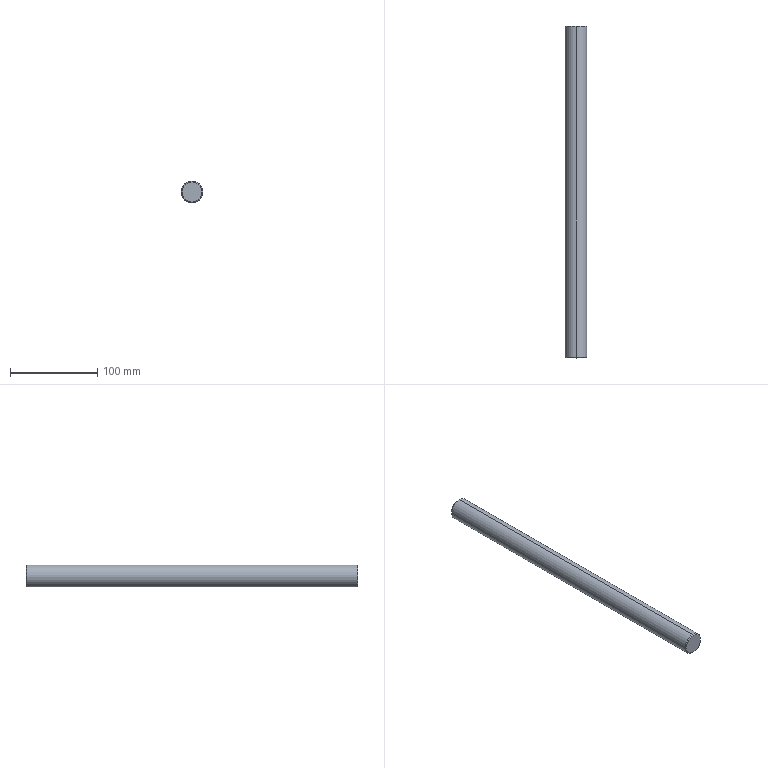Component | SolidWorks | 8TC-A15004-90-02A-1 | 1 solid | 8 faces | box 25 x 380 x 25 mm | volume 186456 mm3 | cone 4 | cylinder 2 | plane 2 | commonest cylinder face diameters 25 x2 | material Chrome Plated Rod
build123d program:
from build123d import *

# Parameters (mm, degrees)
SKETCH1_R           = 12.5
BOSS_EXTRUDE1_DEPTH = 190
CHAMFER1_SIZE       = 1


with BuildPart() as part:
    # Sketch1 → Boss-Extrude1 (new, symmetric)
    with BuildSketch(Plane(origin=(0, 0, 0), x_dir=(0, 0, -1), z_dir=(1, 0, 0))):
        Circle(SKETCH1_R)
    extrude(amount=BOSS_EXTRUDE1_DEPTH, both=True)

    # Chamfer1
    chamfer1_edges = [part.edges().sort_by_distance(p)[0] for p in [
        (-190, 0, 12.5),
        (190, 0, 12.5),
    ]]
    chamfer(chamfer1_edges, length=CHAMFER1_SIZE)


solid = part.part

# Placed as in the assembly
solid = solid.moved(Location((-15, 180, 0), (0, 0, 90)))
STEP:
#1=COLOUR_RGB('',0.7922,0.8196,0.9333);
#2=FILL_AREA_STYLE_COLOUR('',#1);
#3=FILL_AREA_STYLE('',(#2));
#4=SURFACE_STYLE_FILL_AREA(#3);
#5=SURFACE_SIDE_STYLE('',(#4));
#6=SURFACE_STYLE_USAGE(.BOTH.,#5);
#7=PRESENTATION_STYLE_ASSIGNMENT((#6));
#8=CARTESIAN_POINT('',(-0.5906,-0.3937,-0.4528));
#9=VERTEX_POINT('',#8);
#10=CARTESIAN_POINT('',(-0.5906,-0.3937,0.4528));
#11=VERTEX_POINT('',#10);
#12=CARTESIAN_POINT('',(-0.5906,-0.3937,0.));
#13=DIRECTION('',(0.,-1.,0.));
#14=DIRECTION('',(0.,0.,-1.));
#15=AXIS2_PLACEMENT_3D('',#12,#13,#14);
#16=CIRCLE('',#15,0.4528);
#17=EDGE_CURVE('',#9,#11,#16,.T.);
#18=ORIENTED_EDGE('',*,*,#17,.F.);
#19=CARTESIAN_POINT('',(-0.5906,-0.3543,-0.4921));
#20=VERTEX_POINT('',#19);
#21=CARTESIAN_POINT('',(-0.5906,-0.3937,-0.4528));
#22=DIRECTION('',(0.,0.7071,-0.7071));
#23=VECTOR('',#22,39.37);
#24=LINE('',#21,#23);
#25=EDGE_CURVE('',#9,#20,#24,.T.);
#26=ORIENTED_EDGE('',*,*,#25,.T.);
#27=CARTESIAN_POINT('',(-0.5906,-0.3543,0.4921));
#28=VERTEX_POINT('',#27);
#29=CARTESIAN_POINT('',(-0.5906,-0.3543,0.));
#30=DIRECTION('',(0.,1.,0.));
#31=DIRECTION('',(0.,0.,-1.));
#32=AXIS2_PLACEMENT_3D('',#29,#30,#31);
#33=CIRCLE('',#32,0.4921);
#34=EDGE_CURVE('',#28,#20,#33,.T.);
#35=ORIENTED_EDGE('',*,*,#34,.F.);
#36=CARTESIAN_POINT('',(-0.5906,-0.3937,0.4528));
#37=DIRECTION('',(0.,0.7071,0.7071));
#38=VECTOR('',#37,39.37);
#39=LINE('',#36,#38);
#40=EDGE_CURVE('',#11,#28,#39,.T.);
#41=ORIENTED_EDGE('',*,*,#40,.F.);
#42=EDGE_LOOP('',(#18,#26,#35,#41));
#43=FACE_OUTER_BOUND('',#42,.T.);
#44=CARTESIAN_POINT('',(-0.5906,-0.3937,0.));
#45=DIRECTION('',(0.,1.,0.));
#46=DIRECTION('',(0.,0.,1.));
#47=AXIS2_PLACEMENT_3D('',#44,#45,#46);
#48=CONICAL_SURFACE('',#47,0.4528,0.7854);
#49=ADVANCED_FACE('',(#43),#48,.T.);
#50=CARTESIAN_POINT('',(-0.5906,14.567,0.4528));
#51=VERTEX_POINT('',#50);
#52=CARTESIAN_POINT('',(-0.5906,14.567,-0.4528));
#53=VERTEX_POINT('',#52);
#54=CARTESIAN_POINT('',(-0.5906,14.567,0.));
#55=DIRECTION('',(0.,1.,0.));
#56=DIRECTION('',(0.,0.,-1.));
#57=AXIS2_PLACEMENT_3D('',#54,#55,#56);
#58=CIRCLE('',#57,0.4528);
#59=EDGE_CURVE('',#51,#53,#58,.T.);
#60=ORIENTED_EDGE('',*,*,#59,.F.);
#61=CARTESIAN_POINT('',(-0.5906,14.528,0.4921));
#62=VERTEX_POINT('',#61);
#63=CARTESIAN_POINT('',(-0.5906,14.528,0.4921));
#64=DIRECTION('',(0.,-0.7071,0.7071));
#65=VECTOR('',#64,39.37);
#66=LINE('',#63,#65);
#67=EDGE_CURVE('',#51,#62,#66,.T.);
#68=ORIENTED_EDGE('',*,*,#67,.T.);
#69=CARTESIAN_POINT('',(-0.5906,14.528,-0.4921));
#70=VERTEX_POINT('',#69);
#71=CARTESIAN_POINT('',(-0.5906,14.528,0.));
#72=DIRECTION('',(0.,-1.,0.));
#73=DIRECTION('',(0.,0.,-1.));
#74=AXIS2_PLACEMENT_3D('',#71,#72,#73);
#75=CIRCLE('',#74,0.4921);
#76=EDGE_CURVE('',#70,#62,#75,.T.);
#77=ORIENTED_EDGE('',*,*,#76,.F.);
#78=CARTESIAN_POINT('',(-0.5906,14.528,-0.4921));
#79=DIRECTION('',(0.,-0.7071,-0.7071));
#80=VECTOR('',#79,39.37);
#81=LINE('',#78,#80);
#82=EDGE_CURVE('',#53,#70,#81,.T.);
#83=ORIENTED_EDGE('',*,*,#82,.F.);
#84=EDGE_LOOP('',(#60,#68,#77,#83));
#85=FACE_OUTER_BOUND('',#84,.T.);
#86=CARTESIAN_POINT('',(-0.5906,14.528,0.));
#87=DIRECTION('',(0.,-1.,0.));
#88=DIRECTION('',(0.,0.,-1.));
#89=AXIS2_PLACEMENT_3D('',#86,#87,#88);
#90=CONICAL_SURFACE('',#89,0.4921,0.7854);
#91=ADVANCED_FACE('',(#85),#90,.T.);
#92=ORIENTED_EDGE('',*,*,#34,.T.);
#93=CARTESIAN_POINT('',(-0.5906,-0.3937,-0.4921));
#94=DIRECTION('',(0.,1.,0.));
#95=VECTOR('',#94,39.37);
#96=LINE('',#93,#95);
#97=EDGE_CURVE('',#20,#70,#96,.T.);
#98=ORIENTED_EDGE('',*,*,#97,.T.);
#99=ORIENTED_EDGE('',*,*,#76,.T.);
#100=CARTESIAN_POINT('',(-0.5906,-0.3937,0.4921));
#101=DIRECTION('',(0.,1.,0.));
#102=VECTOR('',#101,39.37);
#103=LINE('',#100,#102);
#104=EDGE_CURVE('',#28,#62,#103,.T.);
#105=ORIENTED_EDGE('',*,*,#104,.F.);
#106=EDGE_LOOP('',(#92,#98,#99,#105));
#107=FACE_OUTER_BOUND('',#106,.T.);
#108=CARTESIAN_POINT('',(-0.5906,-0.3937,0.));
#109=DIRECTION('',(0.,1.,0.));
#110=DIRECTION('',(0.,0.,1.));
#111=AXIS2_PLACEMENT_3D('',#108,#109,#110);
#112=CYLINDRICAL_SURFACE('',#111,0.4921);
#113=ADVANCED_FACE('',(#107),#112,.T.);
#114=ORIENTED_EDGE('',*,*,#97,.F.);
#115=CARTESIAN_POINT('',(-0.5906,-0.3543,0.));
#116=DIRECTION('',(0.,1.,0.));
#117=DIRECTION('',(0.,0.,-1.));
#118=AXIS2_PLACEMENT_3D('',#115,#116,#117);
#119=CIRCLE('',#118,0.4921);
#120=EDGE_CURVE('',#20,#28,#119,.T.);
#121=ORIENTED_EDGE('',*,*,#120,.T.);
#122=ORIENTED_EDGE('',*,*,#104,.T.);
#123=CARTESIAN_POINT('',(-0.5906,14.528,0.));
#124=DIRECTION('',(0.,-1.,0.));
#125=DIRECTION('',(0.,0.,-1.));
#126=AXIS2_PLACEMENT_3D('',#123,#124,#125);
#127=CIRCLE('',#126,0.4921);
#128=EDGE_CURVE('',#62,#70,#127,.T.);
#129=ORIENTED_EDGE('',*,*,#128,.T.);
#130=EDGE_LOOP('',(#114,#121,#122,#129));
#131=FACE_OUTER_BOUND('',#130,.T.);
#132=CARTESIAN_POINT('',(-0.5906,-0.3937,0.));
#133=DIRECTION('',(0.,1.,0.));
#134=DIRECTION('',(0.,0.,1.));
#135=AXIS2_PLACEMENT_3D('',#132,#133,#134);
#136=CYLINDRICAL_SURFACE('',#135,0.4921);
#137=ADVANCED_FACE('',(#131),#136,.T.);
#138=CARTESIAN_POINT('',(-0.5906,-0.3937,0.));
#139=DIRECTION('',(0.,-1.,0.));
#140=DIRECTION('',(0.,0.,-1.));
#141=AXIS2_PLACEMENT_3D('',#138,#139,#140);
#142=CIRCLE('',#141,0.4528);
#143=EDGE_CURVE('',#11,#9,#142,.T.);
#144=ORIENTED_EDGE('',*,*,#143,.T.);
#145=ORIENTED_EDGE('',*,*,#17,.T.);
#146=EDGE_LOOP('',(#144,#145));
#147=FACE_OUTER_BOUND('',#146,.T.);
#148=CARTESIAN_POINT('',(-0.5906,-0.3937,0.));
#149=DIRECTION('',(0.,-1.,0.));
#150=DIRECTION('',(0.,0.,-1.));
#151=AXIS2_PLACEMENT_3D('',#148,#149,#150);
#152=PLANE('',#151);
#153=ADVANCED_FACE('',(#147),#152,.T.);
#154=CARTESIAN_POINT('',(-0.5906,14.567,0.));
#155=DIRECTION('',(0.,1.,0.));
#156=DIRECTION('',(0.,0.,-1.));
#157=AXIS2_PLACEMENT_3D('',#154,#155,#156);
#158=CIRCLE('',#157,0.4528);
#159=EDGE_CURVE('',#53,#51,#158,.T.);
#160=ORIENTED_EDGE('',*,*,#159,.T.);
#161=ORIENTED_EDGE('',*,*,#59,.T.);
#162=EDGE_LOOP('',(#160,#161));
#163=FACE_OUTER_BOUND('',#162,.T.);
#164=CARTESIAN_POINT('',(-0.5906,14.567,0.));
#165=DIRECTION('',(0.,-1.,0.));
#166=DIRECTION('',(0.,0.,-1.));
#167=AXIS2_PLACEMENT_3D('',#164,#165,#166);
#168=PLANE('',#167);
#169=ADVANCED_FACE('',(#163),#168,.F.);
#170=ORIENTED_EDGE('',*,*,#67,.F.);
#171=ORIENTED_EDGE('',*,*,#159,.F.);
#172=ORIENTED_EDGE('',*,*,#82,.T.);
#173=ORIENTED_EDGE('',*,*,#128,.F.);
#174=EDGE_LOOP('',(#170,#171,#172,#173));
#175=FACE_OUTER_BOUND('',#174,.T.);
#176=CARTESIAN_POINT('',(-0.5906,14.528,0.));
#177=DIRECTION('',(0.,-1.,0.));
#178=DIRECTION('',(0.,0.,-1.));
#179=AXIS2_PLACEMENT_3D('',#176,#177,#178);
#180=CONICAL_SURFACE('',#179,0.4921,0.7854);
#181=ADVANCED_FACE('',(#175),#180,.T.);
#182=ORIENTED_EDGE('',*,*,#25,.F.);
#183=ORIENTED_EDGE('',*,*,#143,.F.);
#184=ORIENTED_EDGE('',*,*,#40,.T.);
#185=ORIENTED_EDGE('',*,*,#120,.F.);
#186=EDGE_LOOP('',(#182,#183,#184,#185));
#187=FACE_OUTER_BOUND('',#186,.T.);
#188=CARTESIAN_POINT('',(-0.5906,-0.3937,0.));
#189=DIRECTION('',(0.,1.,0.));
#190=DIRECTION('',(0.,0.,1.));
#191=AXIS2_PLACEMENT_3D('',#188,#189,#190);
#192=CONICAL_SURFACE('',#191,0.4528,0.7854);
#193=ADVANCED_FACE('',(#187),#192,.T.);
#194=CLOSED_SHELL('',(#49,#91,#113,#137,#153,#169,#181,#193));
#195=MANIFOLD_SOLID_BREP('',#194);
#196=STYLED_ITEM('',(#7),#195);
#197=PRESENTATION_LAYER_ASSIGNMENT('','',(#196));
#198=CARTESIAN_POINT('',(0.,0.,0.));
#199=DIRECTION('',(0.,0.,1.));
#200=DIRECTION('',(1.,0.,0.));
#201=AXIS2_PLACEMENT_3D('',#198,#199,#200);
#202=(LENGTH_UNIT()NAMED_UNIT(*)SI_UNIT($,.METRE.));
#203=LENGTH_MEASURE_WITH_UNIT(LENGTH_MEASURE(0.0254),#202);
#204=DIMENSIONAL_EXPONENTS(1.,0.,0.,0.,0.,0.,0.);
#205=(CONVERSION_BASED_UNIT('',#203)LENGTH_UNIT()NAMED_UNIT(#204));
#206=UNCERTAINTY_MEASURE_WITH_UNIT(LENGTH_MEASURE(0.00001),#205,'','');
#207=(NAMED_UNIT(*)PLANE_ANGLE_UNIT()SI_UNIT($,.RADIAN.));
#208=(NAMED_UNIT(*)SI_UNIT($,.STERADIAN.)SOLID_ANGLE_UNIT());
#209=(GEOMETRIC_REPRESENTATION_CONTEXT(3)GLOBAL_UNCERTAINTY_ASSIGNED_CONTEXT((#206))GLOBAL_UNIT_ASSIGNED_CONTEXT((#205,#207,#208))REPRESENTATION_CONTEXT('',''));
#210=ADVANCED_BREP_SHAPE_REPRESENTATION('',(#195,#201),#209);
#211=(LENGTH_UNIT()NAMED_UNIT(*)SI_UNIT($,.METRE.));
#212=LENGTH_MEASURE_WITH_UNIT(LENGTH_MEASURE(0.0254),#211);
#213=DIMENSIONAL_EXPONENTS(1.,0.,0.,0.,0.,0.,0.);
#214=(CONVERSION_BASED_UNIT('',#212)LENGTH_UNIT()NAMED_UNIT(#213));
#215=UNCERTAINTY_MEASURE_WITH_UNIT(LENGTH_MEASURE(0.00001),#214,'','');
#216=(NAMED_UNIT(*)PLANE_ANGLE_UNIT()SI_UNIT($,.RADIAN.));
#217=(NAMED_UNIT(*)SI_UNIT($,.STERADIAN.)SOLID_ANGLE_UNIT());
#218=(GEOMETRIC_REPRESENTATION_CONTEXT(3)GLOBAL_UNCERTAINTY_ASSIGNED_CONTEXT((#215))GLOBAL_UNIT_ASSIGNED_CONTEXT((#214,#216,#217))REPRESENTATION_CONTEXT('',''));
#219=MECHANICAL_DESIGN_GEOMETRIC_PRESENTATION_REPRESENTATION('',(#196),#218);